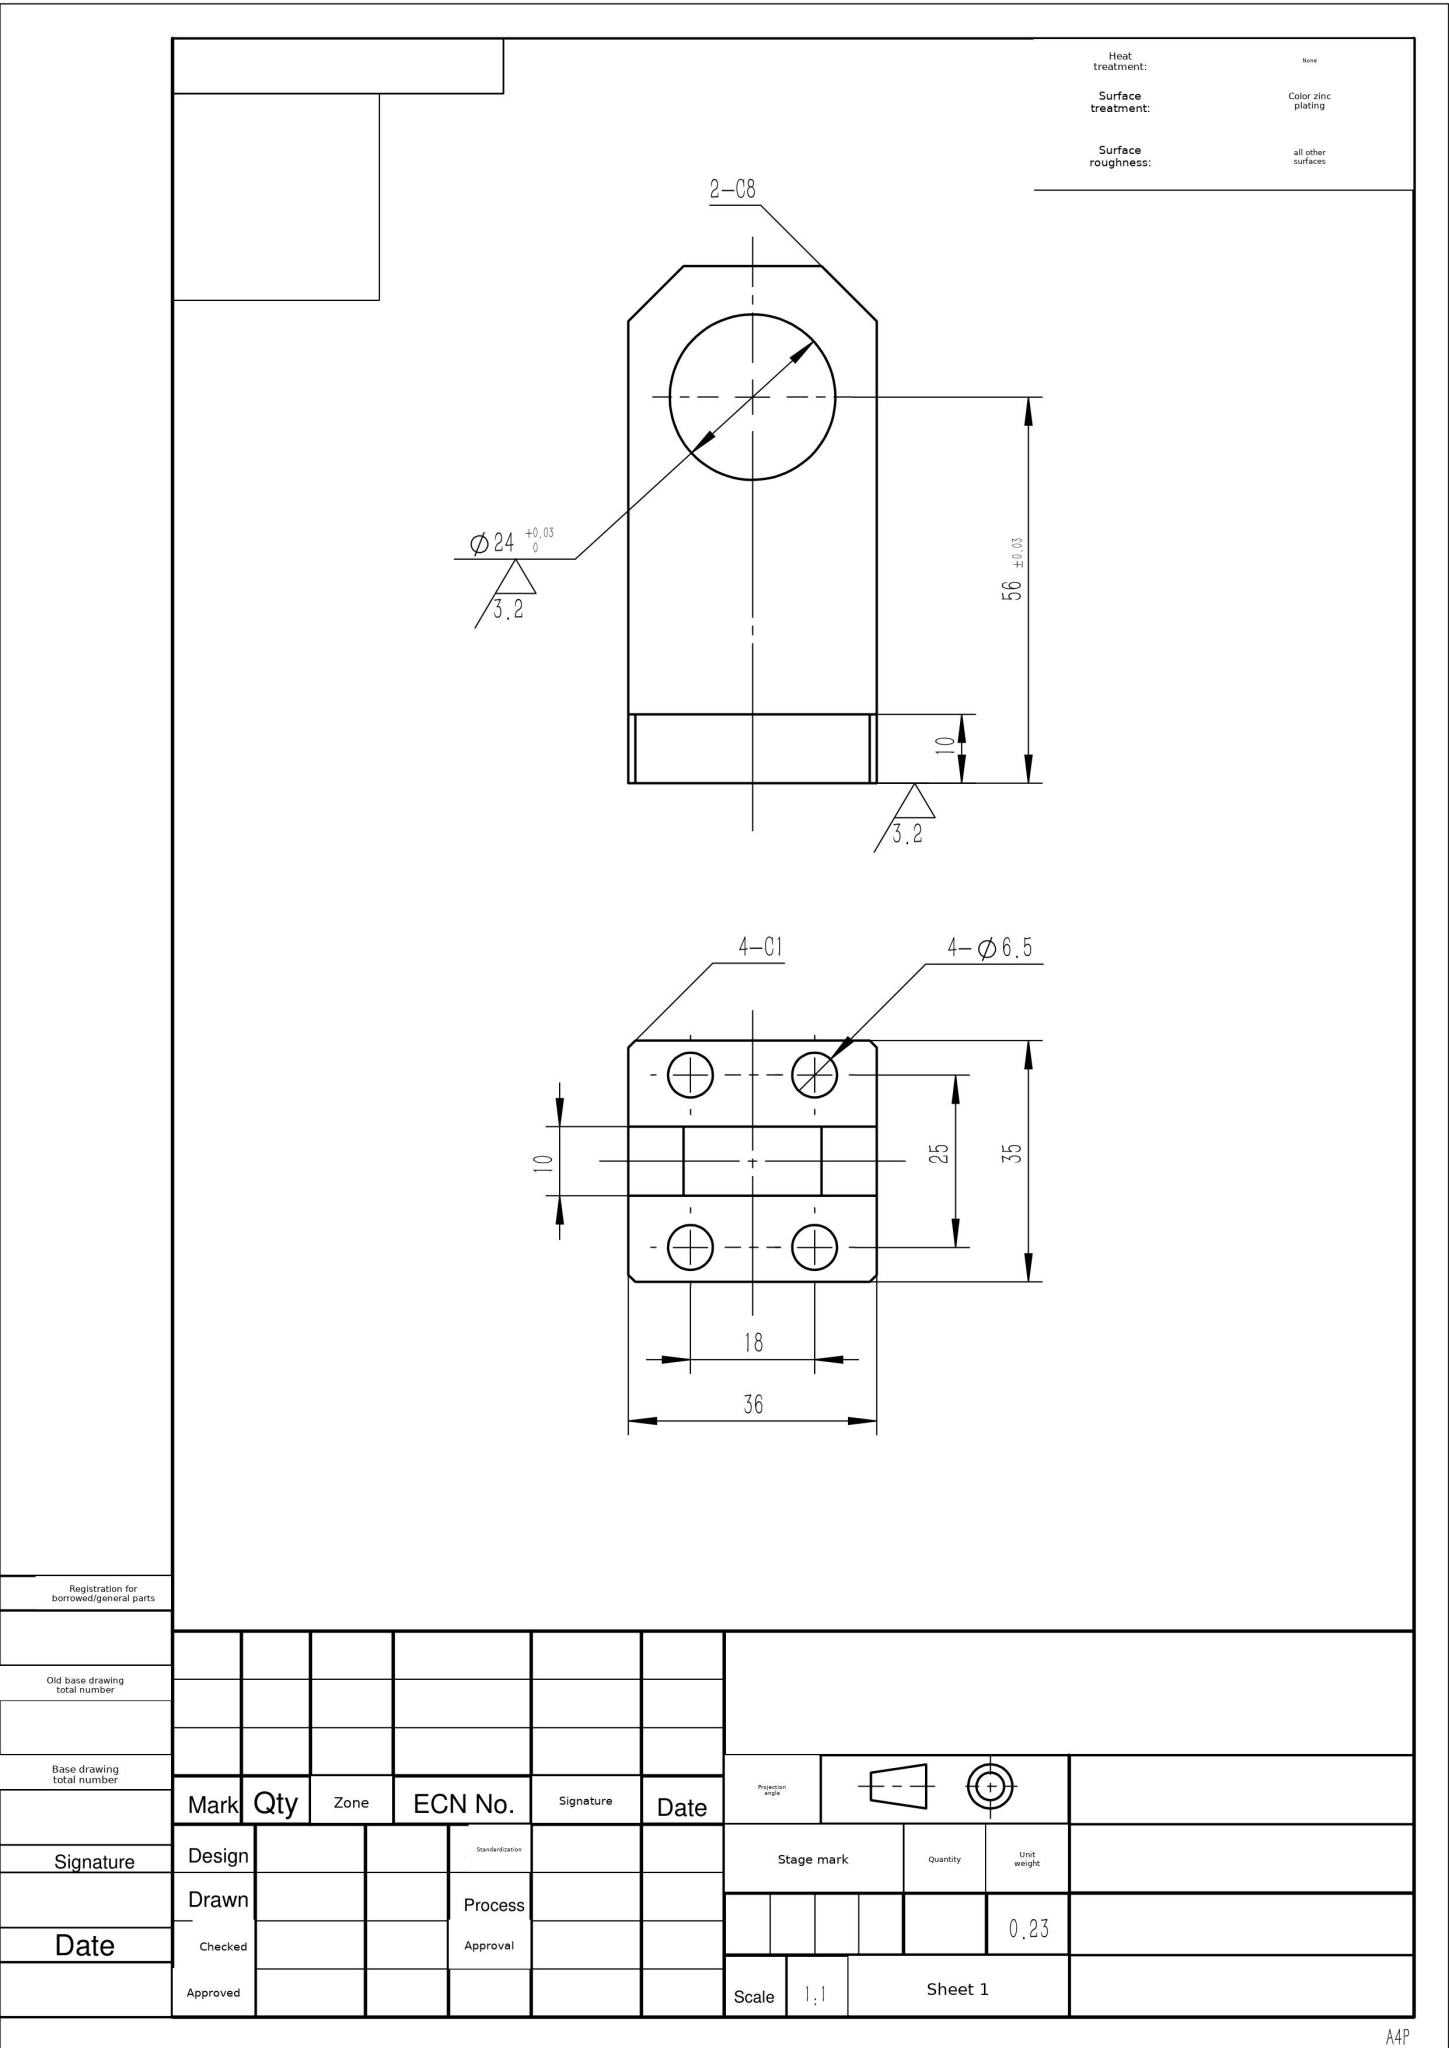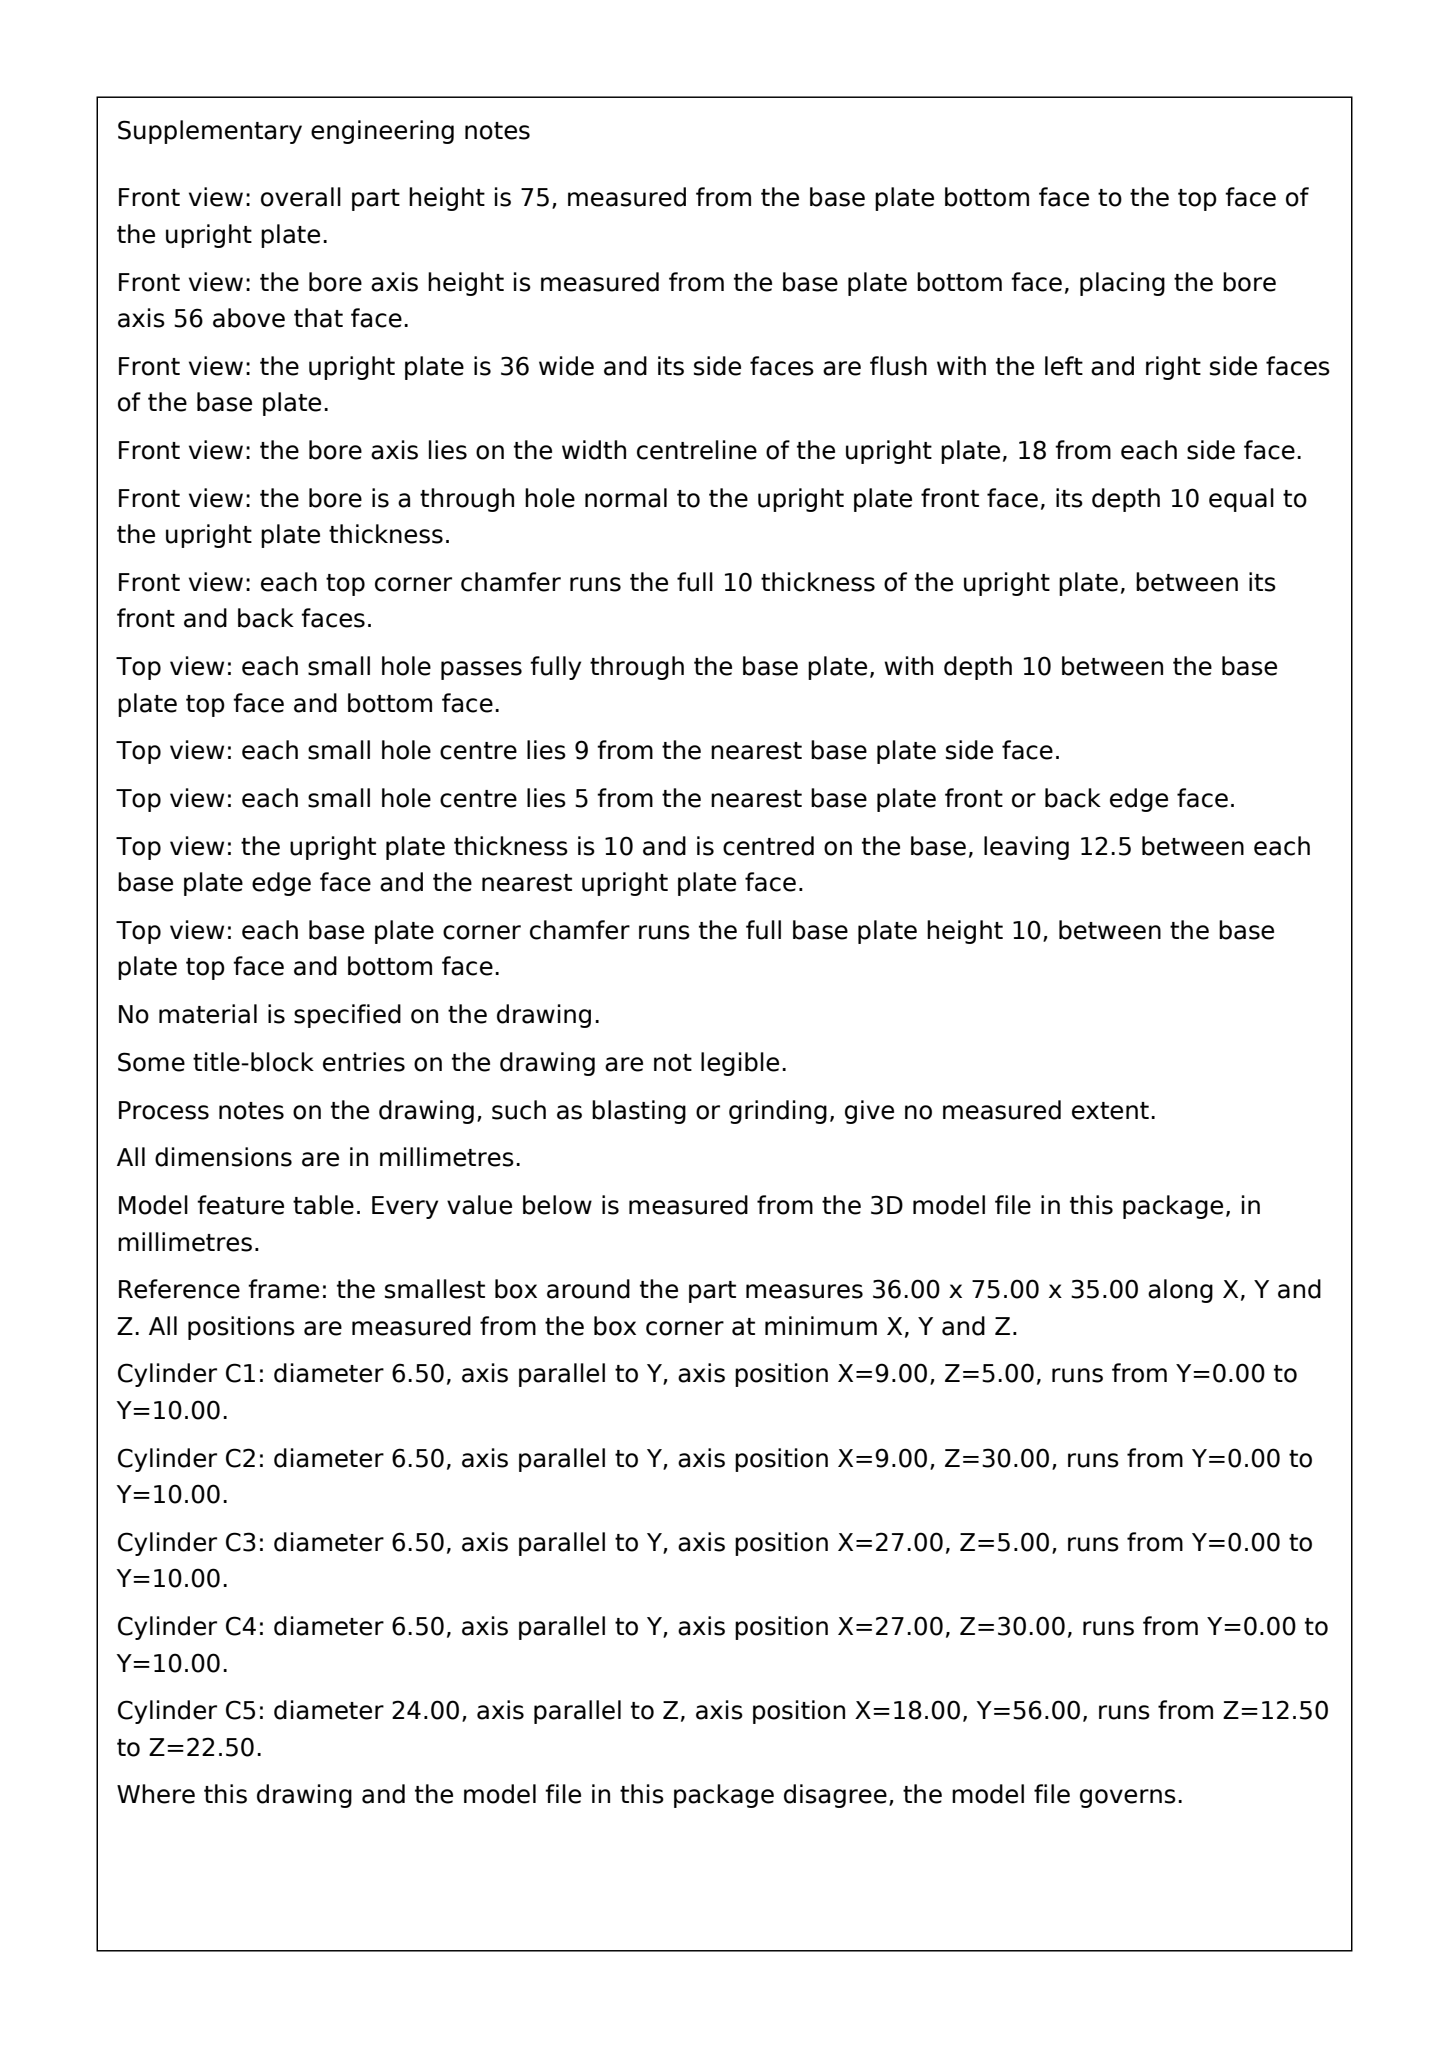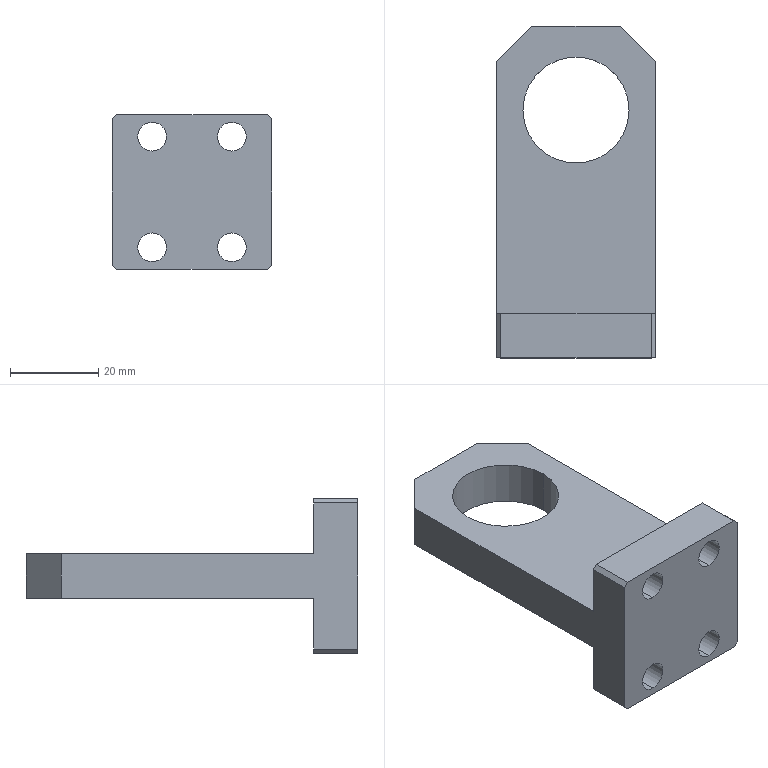Part | SolidWorks | mm | 1 solid | 26 faces | box 36 x 75 x 35 mm | volume 29489 mm3 | plane 16 | cylinder 10 | commonest cylinder face diameters 6.5 x8 24 x2
Drawing notes:
FRONT VIEW: OVERALL HT 75 FROM BOTTOM FACE TO TOP | from the solid: bbox_xyz Y=75; planes y=0 and y=75; hole axis at y=56
OVERALL HT 75 FROM BOTTOM FACE TO TOP OF Ø24 BOSS | from the solid: bbox_xyz y=75; base face y=0, top face plane y=75; Ø24 hole axis at y=56
build123d program:
from build123d import *

# Parameters (mm, degrees)
SKETCH1_W           = 36
SKETCH1_H           = 65
BOSS_EXTRUDE1_DEPTH = 5
SKETCH2_W           = 36
SKETCH2_H           = 35
BOSS_EXTRUDE2_DEPTH = 10
SKETCH3_R           = 12
CUT_EXTRUDE1_DEPTH  = 72.1
CHAMFER1_SIZE       = 8
SKETCH4_R           = 3.25
CUT_EXTRUDE2_DEPTH  = 70.68
CHAMFER2_SIZE       = 1


with BuildPart() as part:
    # Sketch1 → Boss-Extrude1 (new, symmetric)
    with BuildSketch(Plane.XY):
        with Locations((0, 32.5)):
            Rectangle(SKETCH1_W, SKETCH1_H)
    extrude(amount=BOSS_EXTRUDE1_DEPTH, both=True)

    # Sketch2 → Boss-Extrude2 (add)
    with BuildSketch(Plane.XZ):
        Rectangle(SKETCH2_W, SKETCH2_H)
    extrude(amount=BOSS_EXTRUDE2_DEPTH)

    # Sketch3 → Cut-Extrude1 (cut, through all)
    with BuildSketch(Plane(origin=(0, 0, -5), x_dir=(-1, 0, 0), z_dir=(0, 0, -1))):
        with Locations((0, 46)):
            Circle(SKETCH3_R)
    extrude(amount=-CUT_EXTRUDE1_DEPTH, mode=Mode.SUBTRACT)

    # Chamfer1
    chamfer1_edges = [part.edges().sort_by_distance(p)[0] for p in [
        (-18, 65, 0),
        (18, 65, 0),
    ]]
    chamfer(chamfer1_edges, length=CHAMFER1_SIZE)

    # Sketch4 → Cut-Extrude2 (cut, through all)
    with BuildSketch(Plane(origin=(0, 0, 0), x_dir=(1, 0, 0), z_dir=(0, 1, 0))):
        with Locations(Location((-9, -12.5, 0), (0, 0, 270))):
            Circle(SKETCH4_R)
        with Locations(Location((-9, 12.5, 0), (0, 0, 90))):
            Circle(SKETCH4_R)
        with Locations(Location((9, -12.5, 0), (0, 0, 270))):
            Circle(SKETCH4_R)
        with Locations(Location((9, 12.5, 0), (0, 0, 90))):
            Circle(SKETCH4_R)
    extrude(amount=-CUT_EXTRUDE2_DEPTH, mode=Mode.SUBTRACT)

    # Chamfer2
    chamfer2_edges = [part.edges().sort_by_distance(p)[0] for p in [
        (18, -5, -17.5),
        (18, -5, 17.5),
        (-18, -5, 17.5),
        (-18, -5, -17.5),
    ]]
    chamfer(chamfer2_edges, length=CHAMFER2_SIZE)


solid = part.part
STEP:
#1=CARTESIAN_POINT('',(9.,-10.,9.25));
#2=VERTEX_POINT('',#1);
#3=CARTESIAN_POINT('',(9.,-10.,15.75));
#4=VERTEX_POINT('',#3);
#5=CARTESIAN_POINT('',(9.,-10.,12.5));
#6=DIRECTION('',(0.,1.,0.));
#7=DIRECTION('',(0.,0.,1.));
#8=AXIS2_PLACEMENT_3D('',#5,#6,#7);
#9=CIRCLE('',#8,3.25);
#10=EDGE_CURVE('',#2,#4,#9,.T.);
#11=ORIENTED_EDGE('',*,*,#10,.F.);
#12=CARTESIAN_POINT('',(9.,0.,9.25));
#13=VERTEX_POINT('',#12);
#14=CARTESIAN_POINT('',(9.,-10.,9.25));
#15=DIRECTION('',(0.,1.,0.));
#16=VECTOR('',#15,1000.);
#17=LINE('',#14,#16);
#18=EDGE_CURVE('',#2,#13,#17,.T.);
#19=ORIENTED_EDGE('',*,*,#18,.T.);
#20=CARTESIAN_POINT('',(9.,0.,15.75));
#21=VERTEX_POINT('',#20);
#22=CARTESIAN_POINT('',(9.,0.,12.5));
#23=DIRECTION('',(0.,1.,0.));
#24=DIRECTION('',(0.,0.,1.));
#25=AXIS2_PLACEMENT_3D('',#22,#23,#24);
#26=CIRCLE('',#25,3.25);
#27=EDGE_CURVE('',#13,#21,#26,.T.);
#28=ORIENTED_EDGE('',*,*,#27,.T.);
#29=CARTESIAN_POINT('',(9.,-10.,15.75));
#30=DIRECTION('',(0.,1.,0.));
#31=VECTOR('',#30,1000.);
#32=LINE('',#29,#31);
#33=EDGE_CURVE('',#4,#21,#32,.T.);
#34=ORIENTED_EDGE('',*,*,#33,.F.);
#35=EDGE_LOOP('',(#11,#19,#28,#34));
#36=FACE_OUTER_BOUND('',#35,.T.);
#37=CARTESIAN_POINT('',(9.,-10.,12.5));
#38=DIRECTION('',(0.,1.,0.));
#39=DIRECTION('',(0.,0.,1.));
#40=AXIS2_PLACEMENT_3D('',#37,#38,#39);
#41=CYLINDRICAL_SURFACE('',#40,3.25);
#42=ADVANCED_FACE('',(#36),#41,.F.);
#43=CARTESIAN_POINT('',(-9.,-10.,-15.75));
#44=VERTEX_POINT('',#43);
#45=CARTESIAN_POINT('',(-9.,-10.,-9.25));
#46=VERTEX_POINT('',#45);
#47=CARTESIAN_POINT('',(-9.,-10.,-12.5));
#48=DIRECTION('',(0.,1.,0.));
#49=DIRECTION('',(0.,0.,-1.));
#50=AXIS2_PLACEMENT_3D('',#47,#48,#49);
#51=CIRCLE('',#50,3.25);
#52=EDGE_CURVE('',#44,#46,#51,.T.);
#53=ORIENTED_EDGE('',*,*,#52,.F.);
#54=CARTESIAN_POINT('',(-9.,0.,-15.75));
#55=VERTEX_POINT('',#54);
#56=CARTESIAN_POINT('',(-9.,-10.,-15.75));
#57=DIRECTION('',(0.,1.,0.));
#58=VECTOR('',#57,1000.);
#59=LINE('',#56,#58);
#60=EDGE_CURVE('',#44,#55,#59,.T.);
#61=ORIENTED_EDGE('',*,*,#60,.T.);
#62=CARTESIAN_POINT('',(-9.,0.,-9.25));
#63=VERTEX_POINT('',#62);
#64=CARTESIAN_POINT('',(-9.,0.,-12.5));
#65=DIRECTION('',(0.,1.,0.));
#66=DIRECTION('',(0.,0.,-1.));
#67=AXIS2_PLACEMENT_3D('',#64,#65,#66);
#68=CIRCLE('',#67,3.25);
#69=EDGE_CURVE('',#55,#63,#68,.T.);
#70=ORIENTED_EDGE('',*,*,#69,.T.);
#71=CARTESIAN_POINT('',(-9.,-10.,-9.25));
#72=DIRECTION('',(0.,1.,0.));
#73=VECTOR('',#72,1000.);
#74=LINE('',#71,#73);
#75=EDGE_CURVE('',#46,#63,#74,.T.);
#76=ORIENTED_EDGE('',*,*,#75,.F.);
#77=EDGE_LOOP('',(#53,#61,#70,#76));
#78=FACE_OUTER_BOUND('',#77,.T.);
#79=CARTESIAN_POINT('',(-9.,-10.,-12.5));
#80=DIRECTION('',(0.,1.,0.));
#81=DIRECTION('',(0.,0.,1.));
#82=AXIS2_PLACEMENT_3D('',#79,#80,#81);
#83=CYLINDRICAL_SURFACE('',#82,3.25);
#84=ADVANCED_FACE('',(#78),#83,.F.);
#85=CARTESIAN_POINT('',(9.,-10.,-15.75));
#86=VERTEX_POINT('',#85);
#87=CARTESIAN_POINT('',(9.,-10.,-9.25));
#88=VERTEX_POINT('',#87);
#89=CARTESIAN_POINT('',(9.,-10.,-12.5));
#90=DIRECTION('',(0.,1.,0.));
#91=DIRECTION('',(0.,0.,-1.));
#92=AXIS2_PLACEMENT_3D('',#89,#90,#91);
#93=CIRCLE('',#92,3.25);
#94=EDGE_CURVE('',#86,#88,#93,.T.);
#95=ORIENTED_EDGE('',*,*,#94,.F.);
#96=CARTESIAN_POINT('',(9.,0.,-15.75));
#97=VERTEX_POINT('',#96);
#98=CARTESIAN_POINT('',(9.,-10.,-15.75));
#99=DIRECTION('',(0.,1.,0.));
#100=VECTOR('',#99,1000.);
#101=LINE('',#98,#100);
#102=EDGE_CURVE('',#86,#97,#101,.T.);
#103=ORIENTED_EDGE('',*,*,#102,.T.);
#104=CARTESIAN_POINT('',(9.,0.,-9.25));
#105=VERTEX_POINT('',#104);
#106=CARTESIAN_POINT('',(9.,0.,-12.5));
#107=DIRECTION('',(0.,1.,0.));
#108=DIRECTION('',(0.,0.,-1.));
#109=AXIS2_PLACEMENT_3D('',#106,#107,#108);
#110=CIRCLE('',#109,3.25);
#111=EDGE_CURVE('',#97,#105,#110,.T.);
#112=ORIENTED_EDGE('',*,*,#111,.T.);
#113=CARTESIAN_POINT('',(9.,-10.,-9.25));
#114=DIRECTION('',(0.,1.,0.));
#115=VECTOR('',#114,1000.);
#116=LINE('',#113,#115);
#117=EDGE_CURVE('',#88,#105,#116,.T.);
#118=ORIENTED_EDGE('',*,*,#117,.F.);
#119=EDGE_LOOP('',(#95,#103,#112,#118));
#120=FACE_OUTER_BOUND('',#119,.T.);
#121=CARTESIAN_POINT('',(9.,-10.,-12.5));
#122=DIRECTION('',(0.,1.,0.));
#123=DIRECTION('',(0.,0.,1.));
#124=AXIS2_PLACEMENT_3D('',#121,#122,#123);
#125=CYLINDRICAL_SURFACE('',#124,3.25);
#126=ADVANCED_FACE('',(#120),#125,.F.);
#127=CARTESIAN_POINT('',(-9.,-10.,9.25));
#128=VERTEX_POINT('',#127);
#129=CARTESIAN_POINT('',(-9.,-10.,15.75));
#130=VERTEX_POINT('',#129);
#131=CARTESIAN_POINT('',(-9.,-10.,12.5));
#132=DIRECTION('',(0.,1.,0.));
#133=DIRECTION('',(0.,0.,1.));
#134=AXIS2_PLACEMENT_3D('',#131,#132,#133);
#135=CIRCLE('',#134,3.25);
#136=EDGE_CURVE('',#128,#130,#135,.T.);
#137=ORIENTED_EDGE('',*,*,#136,.F.);
#138=CARTESIAN_POINT('',(-9.,0.,9.25));
#139=VERTEX_POINT('',#138);
#140=CARTESIAN_POINT('',(-9.,-10.,9.25));
#141=DIRECTION('',(0.,1.,0.));
#142=VECTOR('',#141,1000.);
#143=LINE('',#140,#142);
#144=EDGE_CURVE('',#128,#139,#143,.T.);
#145=ORIENTED_EDGE('',*,*,#144,.T.);
#146=CARTESIAN_POINT('',(-9.,0.,15.75));
#147=VERTEX_POINT('',#146);
#148=CARTESIAN_POINT('',(-9.,0.,12.5));
#149=DIRECTION('',(0.,1.,0.));
#150=DIRECTION('',(0.,0.,1.));
#151=AXIS2_PLACEMENT_3D('',#148,#149,#150);
#152=CIRCLE('',#151,3.25);
#153=EDGE_CURVE('',#139,#147,#152,.T.);
#154=ORIENTED_EDGE('',*,*,#153,.T.);
#155=CARTESIAN_POINT('',(-9.,-10.,15.75));
#156=DIRECTION('',(0.,1.,0.));
#157=VECTOR('',#156,1000.);
#158=LINE('',#155,#157);
#159=EDGE_CURVE('',#130,#147,#158,.T.);
#160=ORIENTED_EDGE('',*,*,#159,.F.);
#161=EDGE_LOOP('',(#137,#145,#154,#160));
#162=FACE_OUTER_BOUND('',#161,.T.);
#163=CARTESIAN_POINT('',(-9.,-10.,12.5));
#164=DIRECTION('',(0.,1.,0.));
#165=DIRECTION('',(0.,0.,1.));
#166=AXIS2_PLACEMENT_3D('',#163,#164,#165);
#167=CYLINDRICAL_SURFACE('',#166,3.25);
#168=ADVANCED_FACE('',(#162),#167,.F.);
#169=CARTESIAN_POINT('',(-12.,46.,5.));
#170=VERTEX_POINT('',#169);
#171=CARTESIAN_POINT('',(12.,46.,5.));
#172=VERTEX_POINT('',#171);
#173=CARTESIAN_POINT('',(0.,46.,5.));
#174=DIRECTION('',(0.,0.,1.));
#175=DIRECTION('',(1.,0.,0.));
#176=AXIS2_PLACEMENT_3D('',#173,#174,#175);
#177=CIRCLE('',#176,12.);
#178=EDGE_CURVE('',#170,#172,#177,.T.);
#179=ORIENTED_EDGE('',*,*,#178,.T.);
#180=CARTESIAN_POINT('',(12.,46.,-5.));
#181=VERTEX_POINT('',#180);
#182=CARTESIAN_POINT('',(12.,46.,17.5));
#183=DIRECTION('',(0.,0.,-1.));
#184=VECTOR('',#183,1000.);
#185=LINE('',#182,#184);
#186=EDGE_CURVE('',#172,#181,#185,.T.);
#187=ORIENTED_EDGE('',*,*,#186,.T.);
#188=CARTESIAN_POINT('',(-12.,46.,-5.));
#189=VERTEX_POINT('',#188);
#190=CARTESIAN_POINT('',(0.,46.,-5.));
#191=DIRECTION('',(0.,0.,-1.));
#192=DIRECTION('',(-1.,0.,0.));
#193=AXIS2_PLACEMENT_3D('',#190,#191,#192);
#194=CIRCLE('',#193,12.);
#195=EDGE_CURVE('',#181,#189,#194,.T.);
#196=ORIENTED_EDGE('',*,*,#195,.T.);
#197=CARTESIAN_POINT('',(-12.,46.,17.5));
#198=DIRECTION('',(0.,0.,-1.));
#199=VECTOR('',#198,1000.);
#200=LINE('',#197,#199);
#201=EDGE_CURVE('',#170,#189,#200,.T.);
#202=ORIENTED_EDGE('',*,*,#201,.F.);
#203=EDGE_LOOP('',(#179,#187,#196,#202));
#204=FACE_OUTER_BOUND('',#203,.T.);
#205=CARTESIAN_POINT('',(0.,46.,17.5));
#206=DIRECTION('',(0.,0.,-1.));
#207=DIRECTION('',(-1.,0.,0.));
#208=AXIS2_PLACEMENT_3D('',#205,#206,#207);
#209=CYLINDRICAL_SURFACE('',#208,12.);
#210=ADVANCED_FACE('',(#204),#209,.F.);
#211=CARTESIAN_POINT('',(-18.,0.,-5.));
#212=VERTEX_POINT('',#211);
#213=CARTESIAN_POINT('',(-18.,0.,-16.5));
#214=VERTEX_POINT('',#213);
#215=CARTESIAN_POINT('',(-18.,0.,-17.5));
#216=DIRECTION('',(0.,0.,-1.));
#217=VECTOR('',#216,1000.);
#218=LINE('',#215,#217);
#219=EDGE_CURVE('',#212,#214,#218,.T.);
#220=ORIENTED_EDGE('',*,*,#219,.T.);
#221=CARTESIAN_POINT('',(-18.,-10.,-16.5));
#222=VERTEX_POINT('',#221);
#223=CARTESIAN_POINT('',(-18.,65.,-16.5));
#224=DIRECTION('',(0.,-1.,0.));
#225=VECTOR('',#224,1000.);
#226=LINE('',#223,#225);
#227=EDGE_CURVE('',#214,#222,#226,.T.);
#228=ORIENTED_EDGE('',*,*,#227,.T.);
#229=CARTESIAN_POINT('',(-18.,-10.,16.5));
#230=VERTEX_POINT('',#229);
#231=CARTESIAN_POINT('',(-18.,-10.,-17.5));
#232=DIRECTION('',(0.,0.,-1.));
#233=VECTOR('',#232,1000.);
#234=LINE('',#231,#233);
#235=EDGE_CURVE('',#230,#222,#234,.T.);
#236=ORIENTED_EDGE('',*,*,#235,.F.);
#237=CARTESIAN_POINT('',(-18.,0.,16.5));
#238=VERTEX_POINT('',#237);
#239=CARTESIAN_POINT('',(-18.,65.,16.5));
#240=DIRECTION('',(-0.,1.,0.));
#241=VECTOR('',#240,1000.);
#242=LINE('',#239,#241);
#243=EDGE_CURVE('',#230,#238,#242,.T.);
#244=ORIENTED_EDGE('',*,*,#243,.T.);
#245=CARTESIAN_POINT('',(-18.,0.,5.));
#246=VERTEX_POINT('',#245);
#247=CARTESIAN_POINT('',(-18.,0.,-17.5));
#248=DIRECTION('',(0.,0.,-1.));
#249=VECTOR('',#248,1000.);
#250=LINE('',#247,#249);
#251=EDGE_CURVE('',#238,#246,#250,.T.);
#252=ORIENTED_EDGE('',*,*,#251,.T.);
#253=CARTESIAN_POINT('',(-18.,57.,5.));
#254=VERTEX_POINT('',#253);
#255=CARTESIAN_POINT('',(-18.,65.,5.));
#256=DIRECTION('',(0.,-1.,0.));
#257=VECTOR('',#256,1000.);
#258=LINE('',#255,#257);
#259=EDGE_CURVE('',#254,#246,#258,.T.);
#260=ORIENTED_EDGE('',*,*,#259,.F.);
#261=CARTESIAN_POINT('',(-18.,57.,-5.));
#262=VERTEX_POINT('',#261);
#263=CARTESIAN_POINT('',(-18.,57.,5.));
#264=DIRECTION('',(0.,0.,-1.));
#265=VECTOR('',#264,1000.);
#266=LINE('',#263,#265);
#267=EDGE_CURVE('',#254,#262,#266,.T.);
#268=ORIENTED_EDGE('',*,*,#267,.T.);
#269=CARTESIAN_POINT('',(-18.,65.,-5.));
#270=DIRECTION('',(0.,-1.,0.));
#271=VECTOR('',#270,1000.);
#272=LINE('',#269,#271);
#273=EDGE_CURVE('',#262,#212,#272,.T.);
#274=ORIENTED_EDGE('',*,*,#273,.T.);
#275=EDGE_LOOP('',(#220,#228,#236,#244,#252,#260,#268,#274));
#276=FACE_OUTER_BOUND('',#275,.T.);
#277=CARTESIAN_POINT('',(-18.,65.,5.));
#278=DIRECTION('',(1.,0.,0.));
#279=DIRECTION('',(-0.,1.,0.));
#280=AXIS2_PLACEMENT_3D('',#277,#278,#279);
#281=PLANE('',#280);
#282=ADVANCED_FACE('',(#276),#281,.F.);
#283=CARTESIAN_POINT('',(18.,-10.,-16.5));
#284=VERTEX_POINT('',#283);
#285=CARTESIAN_POINT('',(18.,-10.,16.5));
#286=VERTEX_POINT('',#285);
#287=CARTESIAN_POINT('',(18.,-10.,-17.5));
#288=DIRECTION('',(0.,0.,1.));
#289=VECTOR('',#288,1000.);
#290=LINE('',#287,#289);
#291=EDGE_CURVE('',#284,#286,#290,.T.);
#292=ORIENTED_EDGE('',*,*,#291,.F.);
#293=CARTESIAN_POINT('',(18.,0.,-16.5));
#294=VERTEX_POINT('',#293);
#295=CARTESIAN_POINT('',(18.,65.,-16.5));
#296=DIRECTION('',(0.,1.,0.));
#297=VECTOR('',#296,1000.);
#298=LINE('',#295,#297);
#299=EDGE_CURVE('',#284,#294,#298,.T.);
#300=ORIENTED_EDGE('',*,*,#299,.T.);
#301=CARTESIAN_POINT('',(18.,0.,-5.));
#302=VERTEX_POINT('',#301);
#303=CARTESIAN_POINT('',(18.,0.,-17.5));
#304=DIRECTION('',(0.,0.,1.));
#305=VECTOR('',#304,1000.);
#306=LINE('',#303,#305);
#307=EDGE_CURVE('',#294,#302,#306,.T.);
#308=ORIENTED_EDGE('',*,*,#307,.T.);
#309=CARTESIAN_POINT('',(18.,57.,-5.));
#310=VERTEX_POINT('',#309);
#311=CARTESIAN_POINT('',(18.,65.,-5.));
#312=DIRECTION('',(0.,1.,0.));
#313=VECTOR('',#312,1000.);
#314=LINE('',#311,#313);
#315=EDGE_CURVE('',#302,#310,#314,.T.);
#316=ORIENTED_EDGE('',*,*,#315,.T.);
#317=CARTESIAN_POINT('',(18.,57.,5.));
#318=VERTEX_POINT('',#317);
#319=CARTESIAN_POINT('',(18.,57.,5.));
#320=DIRECTION('',(0.,0.,1.));
#321=VECTOR('',#320,1000.);
#322=LINE('',#319,#321);
#323=EDGE_CURVE('',#310,#318,#322,.T.);
#324=ORIENTED_EDGE('',*,*,#323,.T.);
#325=CARTESIAN_POINT('',(18.,0.,5.));
#326=VERTEX_POINT('',#325);
#327=CARTESIAN_POINT('',(18.,65.,5.));
#328=DIRECTION('',(0.,1.,0.));
#329=VECTOR('',#328,1000.);
#330=LINE('',#327,#329);
#331=EDGE_CURVE('',#326,#318,#330,.T.);
#332=ORIENTED_EDGE('',*,*,#331,.F.);
#333=CARTESIAN_POINT('',(18.,0.,16.5));
#334=VERTEX_POINT('',#333);
#335=CARTESIAN_POINT('',(18.,0.,-17.5));
#336=DIRECTION('',(0.,0.,1.));
#337=VECTOR('',#336,1000.);
#338=LINE('',#335,#337);
#339=EDGE_CURVE('',#326,#334,#338,.T.);
#340=ORIENTED_EDGE('',*,*,#339,.T.);
#341=CARTESIAN_POINT('',(18.,65.,16.5));
#342=DIRECTION('',(-0.,-1.,0.));
#343=VECTOR('',#342,1000.);
#344=LINE('',#341,#343);
#345=EDGE_CURVE('',#334,#286,#344,.T.);
#346=ORIENTED_EDGE('',*,*,#345,.T.);
#347=EDGE_LOOP('',(#292,#300,#308,#316,#324,#332,#340,#346));
#348=FACE_OUTER_BOUND('',#347,.T.);
#349=CARTESIAN_POINT('',(18.,65.,5.));
#350=DIRECTION('',(-1.,0.,0.));
#351=DIRECTION('',(-0.,-1.,0.));
#352=AXIS2_PLACEMENT_3D('',#349,#350,#351);
#353=PLANE('',#352);
#354=ADVANCED_FACE('',(#348),#353,.F.);
#355=CARTESIAN_POINT('',(10.,65.,-5.));
#356=VERTEX_POINT('',#355);
#357=CARTESIAN_POINT('',(-10.,65.,-5.));
#358=VERTEX_POINT('',#357);
#359=CARTESIAN_POINT('',(18.,65.,-5.));
#360=DIRECTION('',(-1.,0.,0.));
#361=VECTOR('',#360,1000.);
#362=LINE('',#359,#361);
#363=EDGE_CURVE('',#356,#358,#362,.T.);
#364=ORIENTED_EDGE('',*,*,#363,.T.);
#365=CARTESIAN_POINT('',(-10.,65.,5.));
#366=VERTEX_POINT('',#365);
#367=CARTESIAN_POINT('',(-10.,65.,5.));
#368=DIRECTION('',(0.,0.,1.));
#369=VECTOR('',#368,1000.);
#370=LINE('',#367,#369);
#371=EDGE_CURVE('',#358,#366,#370,.T.);
#372=ORIENTED_EDGE('',*,*,#371,.T.);
#373=CARTESIAN_POINT('',(10.,65.,5.));
#374=VERTEX_POINT('',#373);
#375=CARTESIAN_POINT('',(18.,65.,5.));
#376=DIRECTION('',(-1.,0.,0.));
#377=VECTOR('',#376,1000.);
#378=LINE('',#375,#377);
#379=EDGE_CURVE('',#374,#366,#378,.T.);
#380=ORIENTED_EDGE('',*,*,#379,.F.);
#381=CARTESIAN_POINT('',(10.,65.,5.));
#382=DIRECTION('',(0.,0.,-1.));
#383=VECTOR('',#382,1000.);
#384=LINE('',#381,#383);
#385=EDGE_CURVE('',#374,#356,#384,.T.);
#386=ORIENTED_EDGE('',*,*,#385,.T.);
#387=EDGE_LOOP('',(#364,#372,#380,#386));
#388=FACE_OUTER_BOUND('',#387,.T.);
#389=CARTESIAN_POINT('',(18.,65.,5.));
#390=DIRECTION('',(0.,-1.,0.));
#391=DIRECTION('',(0.,0.,-1.));
#392=AXIS2_PLACEMENT_3D('',#389,#390,#391);
#393=PLANE('',#392);
#394=ADVANCED_FACE('',(#388),#393,.F.);
#395=ORIENTED_EDGE('',*,*,#178,.F.);
#396=CARTESIAN_POINT('',(0.,46.,5.));
#397=DIRECTION('',(0.,0.,1.));
#398=DIRECTION('',(1.,0.,0.));
#399=AXIS2_PLACEMENT_3D('',#396,#397,#398);
#400=CIRCLE('',#399,12.);
#401=EDGE_CURVE('',#172,#170,#400,.T.);
#402=ORIENTED_EDGE('',*,*,#401,.F.);
#403=EDGE_LOOP('',(#395,#402));
#404=FACE_BOUND('',#403,.T.);
#405=ORIENTED_EDGE('',*,*,#379,.T.);
#406=CARTESIAN_POINT('',(-37.5,37.5,5.));
#407=DIRECTION('',(-0.7071,-0.7071,0.));
#408=VECTOR('',#407,1000.);
#409=LINE('',#406,#408);
#410=EDGE_CURVE('',#366,#254,#409,.T.);
#411=ORIENTED_EDGE('',*,*,#410,.T.);
#412=ORIENTED_EDGE('',*,*,#259,.T.);
#413=CARTESIAN_POINT('',(-18.,0.,5.));
#414=DIRECTION('',(1.,0.,0.));
#415=VECTOR('',#414,1000.);
#416=LINE('',#413,#415);
#417=EDGE_CURVE('',#246,#326,#416,.T.);
#418=ORIENTED_EDGE('',*,*,#417,.T.);
#419=ORIENTED_EDGE('',*,*,#331,.T.);
#420=CARTESIAN_POINT('',(37.5,37.5,5.));
#421=DIRECTION('',(-0.7071,0.7071,0.));
#422=VECTOR('',#421,1000.);
#423=LINE('',#420,#422);
#424=EDGE_CURVE('',#318,#374,#423,.T.);
#425=ORIENTED_EDGE('',*,*,#424,.T.);
#426=EDGE_LOOP('',(#405,#411,#412,#418,#419,#425));
#427=FACE_OUTER_BOUND('',#426,.T.);
#428=CARTESIAN_POINT('',(0.,0.,5.));
#429=DIRECTION('',(0.,0.,1.));
#430=DIRECTION('',(1.,0.,0.));
#431=AXIS2_PLACEMENT_3D('',#428,#429,#430);
#432=PLANE('',#431);
#433=ADVANCED_FACE('',(#404,#427),#432,.T.);
#434=CARTESIAN_POINT('',(0.,46.,-5.));
#435=DIRECTION('',(0.,0.,-1.));
#436=DIRECTION('',(-1.,0.,0.));
#437=AXIS2_PLACEMENT_3D('',#434,#435,#436);
#438=CIRCLE('',#437,12.);
#439=EDGE_CURVE('',#189,#181,#438,.T.);
#440=ORIENTED_EDGE('',*,*,#439,.F.);
#441=ORIENTED_EDGE('',*,*,#195,.F.);
#442=EDGE_LOOP('',(#440,#441));
#443=FACE_BOUND('',#442,.T.);
#444=ORIENTED_EDGE('',*,*,#273,.F.);
#445=CARTESIAN_POINT('',(-18.,57.,-5.));
#446=DIRECTION('',(0.7071,0.7071,0.));
#447=VECTOR('',#446,1000.);
#448=LINE('',#445,#447);
#449=EDGE_CURVE('',#262,#358,#448,.T.);
#450=ORIENTED_EDGE('',*,*,#449,.T.);
#451=ORIENTED_EDGE('',*,*,#363,.F.);
#452=CARTESIAN_POINT('',(10.,65.,-5.));
#453=DIRECTION('',(0.7071,-0.7071,0.));
#454=VECTOR('',#453,1000.);
#455=LINE('',#452,#454);
#456=EDGE_CURVE('',#356,#310,#455,.T.);
#457=ORIENTED_EDGE('',*,*,#456,.T.);
#458=ORIENTED_EDGE('',*,*,#315,.F.);
#459=CARTESIAN_POINT('',(-18.,0.,-5.));
#460=DIRECTION('',(1.,0.,0.));
#461=VECTOR('',#460,1000.);
#462=LINE('',#459,#461);
#463=EDGE_CURVE('',#212,#302,#462,.T.);
#464=ORIENTED_EDGE('',*,*,#463,.F.);
#465=EDGE_LOOP('',(#444,#450,#451,#457,#458,#464));
#466=FACE_OUTER_BOUND('',#465,.T.);
#467=CARTESIAN_POINT('',(0.,0.,-5.));
#468=DIRECTION('',(0.,0.,1.));
#469=DIRECTION('',(1.,0.,0.));
#470=AXIS2_PLACEMENT_3D('',#467,#468,#469);
#471=PLANE('',#470);
#472=ADVANCED_FACE('',(#443,#466),#471,.F.);
#473=CARTESIAN_POINT('',(9.,0.,12.5));
#474=DIRECTION('',(0.,1.,0.));
#475=DIRECTION('',(0.,0.,1.));
#476=AXIS2_PLACEMENT_3D('',#473,#474,#475);
#477=CIRCLE('',#476,3.25);
#478=EDGE_CURVE('',#21,#13,#477,.T.);
#479=ORIENTED_EDGE('',*,*,#478,.F.);
#480=ORIENTED_EDGE('',*,*,#27,.F.);
#481=EDGE_LOOP('',(#479,#480));
#482=FACE_BOUND('',#481,.T.);
#483=CARTESIAN_POINT('',(-9.,0.,12.5));
#484=DIRECTION('',(0.,1.,0.));
#485=DIRECTION('',(0.,0.,1.));
#486=AXIS2_PLACEMENT_3D('',#483,#484,#485);
#487=CIRCLE('',#486,3.25);
#488=EDGE_CURVE('',#147,#139,#487,.T.);
#489=ORIENTED_EDGE('',*,*,#488,.F.);
#490=ORIENTED_EDGE('',*,*,#153,.F.);
#491=EDGE_LOOP('',(#489,#490));
#492=FACE_BOUND('',#491,.T.);
#493=ORIENTED_EDGE('',*,*,#251,.F.);
#494=CARTESIAN_POINT('',(-17.,0.,17.5));
#495=VERTEX_POINT('',#494);
#496=CARTESIAN_POINT('',(-17.25,0.,17.25));
#497=DIRECTION('',(0.7071,0.,0.7071));
#498=VECTOR('',#497,1000.);
#499=LINE('',#496,#498);
#500=EDGE_CURVE('',#238,#495,#499,.T.);
#501=ORIENTED_EDGE('',*,*,#500,.T.);
#502=CARTESIAN_POINT('',(17.,0.,17.5));
#503=VERTEX_POINT('',#502);
#504=CARTESIAN_POINT('',(-18.,0.,17.5));
#505=DIRECTION('',(-1.,0.,0.));
#506=VECTOR('',#505,1000.);
#507=LINE('',#504,#506);
#508=EDGE_CURVE('',#503,#495,#507,.T.);
#509=ORIENTED_EDGE('',*,*,#508,.F.);
#510=CARTESIAN_POINT('',(17.25,0.,17.25));
#511=DIRECTION('',(0.7071,0.,-0.7071));
#512=VECTOR('',#511,1000.);
#513=LINE('',#510,#512);
#514=EDGE_CURVE('',#503,#334,#513,.T.);
#515=ORIENTED_EDGE('',*,*,#514,.T.);
#516=ORIENTED_EDGE('',*,*,#339,.F.);
#517=ORIENTED_EDGE('',*,*,#417,.F.);
#518=EDGE_LOOP('',(#493,#501,#509,#515,#516,#517));
#519=FACE_OUTER_BOUND('',#518,.T.);
#520=CARTESIAN_POINT('',(0.,0.,0.));
#521=DIRECTION('',(0.,1.,0.));
#522=DIRECTION('',(0.,0.,1.));
#523=AXIS2_PLACEMENT_3D('',#520,#521,#522);
#524=PLANE('',#523);
#525=ADVANCED_FACE('',(#482,#492,#519),#524,.T.);
#526=ORIENTED_EDGE('',*,*,#508,.T.);
#527=CARTESIAN_POINT('',(-17.,-10.,17.5));
#528=VERTEX_POINT('',#527);
#529=CARTESIAN_POINT('',(-17.,-10.,17.5));
#530=DIRECTION('',(0.,-1.,0.));
#531=VECTOR('',#530,1000.);
#532=LINE('',#529,#531);
#533=EDGE_CURVE('',#495,#528,#532,.T.);
#534=ORIENTED_EDGE('',*,*,#533,.T.);
#535=CARTESIAN_POINT('',(17.,-10.,17.5));
#536=VERTEX_POINT('',#535);
#537=CARTESIAN_POINT('',(-18.,-10.,17.5));
#538=DIRECTION('',(-1.,0.,0.));
#539=VECTOR('',#538,1000.);
#540=LINE('',#537,#539);
#541=EDGE_CURVE('',#536,#528,#540,.T.);
#542=ORIENTED_EDGE('',*,*,#541,.F.);
#543=CARTESIAN_POINT('',(17.,-10.,17.5));
#544=DIRECTION('',(0.,1.,0.));
#545=VECTOR('',#544,1000.);
#546=LINE('',#543,#545);
#547=EDGE_CURVE('',#536,#503,#546,.T.);
#548=ORIENTED_EDGE('',*,*,#547,.T.);
#549=EDGE_LOOP('',(#526,#534,#542,#548));
#550=FACE_OUTER_BOUND('',#549,.T.);
#551=CARTESIAN_POINT('',(-18.,-10.,17.5));
#552=DIRECTION('',(0.,0.,-1.));
#553=DIRECTION('',(-1.,0.,0.));
#554=AXIS2_PLACEMENT_3D('',#551,#552,#553);
#555=PLANE('',#554);
#556=ADVANCED_FACE('',(#550),#555,.F.);
#557=CARTESIAN_POINT('',(-17.,0.,-17.5));
#558=VERTEX_POINT('',#557);
#559=CARTESIAN_POINT('',(17.,0.,-17.5));
#560=VERTEX_POINT('',#559);
#561=CARTESIAN_POINT('',(-18.,0.,-17.5));
#562=DIRECTION('',(1.,0.,0.));
#563=VECTOR('',#562,1000.);
#564=LINE('',#561,#563);
#565=EDGE_CURVE('',#558,#560,#564,.T.);
#566=ORIENTED_EDGE('',*,*,#565,.T.);
#567=CARTESIAN_POINT('',(17.,-10.,-17.5));
#568=VERTEX_POINT('',#567);
#569=CARTESIAN_POINT('',(17.,-10.,-17.5));
#570=DIRECTION('',(-0.,-1.,0.));
#571=VECTOR('',#570,1000.);
#572=LINE('',#569,#571);
#573=EDGE_CURVE('',#560,#568,#572,.T.);
#574=ORIENTED_EDGE('',*,*,#573,.T.);
#575=CARTESIAN_POINT('',(-17.,-10.,-17.5));
#576=VERTEX_POINT('',#575);
#577=CARTESIAN_POINT('',(-18.,-10.,-17.5));
#578=DIRECTION('',(1.,0.,0.));
#579=VECTOR('',#578,1000.);
#580=LINE('',#577,#579);
#581=EDGE_CURVE('',#576,#568,#580,.T.);
#582=ORIENTED_EDGE('',*,*,#581,.F.);
#583=CARTESIAN_POINT('',(-17.,-10.,-17.5));
#584=DIRECTION('',(-0.,1.,0.));
#585=VECTOR('',#584,1000.);
#586=LINE('',#583,#585);
#587=EDGE_CURVE('',#576,#558,#586,.T.);
#588=ORIENTED_EDGE('',*,*,#587,.T.);
#589=EDGE_LOOP('',(#566,#574,#582,#588));
#590=FACE_OUTER_BOUND('',#589,.T.);
#591=CARTESIAN_POINT('',(-18.,-10.,-17.5));
#592=DIRECTION('',(0.,0.,1.));
#593=DIRECTION('',(1.,0.,0.));
#594=AXIS2_PLACEMENT_3D('',#591,#592,#593);
#595=PLANE('',#594);
#596=ADVANCED_FACE('',(#590),#595,.F.);
#597=CARTESIAN_POINT('',(-9.,-10.,-12.5));
#598=DIRECTION('',(0.,1.,0.));
#599=DIRECTION('',(0.,0.,-1.));
#600=AXIS2_PLACEMENT_3D('',#597,#598,#599);
#601=CIRCLE('',#600,3.25);
#602=EDGE_CURVE('',#46,#44,#601,.T.);
#603=ORIENTED_EDGE('',*,*,#602,.T.);
#604=ORIENTED_EDGE('',*,*,#52,.T.);
#605=EDGE_LOOP('',(#603,#604));
#606=FACE_BOUND('',#605,.T.);
#607=CARTESIAN_POINT('',(9.,-10.,12.5));
#608=DIRECTION('',(0.,1.,0.));
#609=DIRECTION('',(0.,0.,1.));
#610=AXIS2_PLACEMENT_3D('',#607,#608,#609);
#611=CIRCLE('',#610,3.25);
#612=EDGE_CURVE('',#4,#2,#611,.T.);
#613=ORIENTED_EDGE('',*,*,#612,.T.);
#614=ORIENTED_EDGE('',*,*,#10,.T.);
#615=EDGE_LOOP('',(#613,#614));
#616=FACE_BOUND('',#615,.T.);
#617=CARTESIAN_POINT('',(9.,-10.,-12.5));
#618=DIRECTION('',(0.,1.,0.));
#619=DIRECTION('',(0.,0.,-1.));
#620=AXIS2_PLACEMENT_3D('',#617,#618,#619);
#621=CIRCLE('',#620,3.25);
#622=EDGE_CURVE('',#88,#86,#621,.T.);
#623=ORIENTED_EDGE('',*,*,#622,.T.);
#624=ORIENTED_EDGE('',*,*,#94,.T.);
#625=EDGE_LOOP('',(#623,#624));
#626=FACE_BOUND('',#625,.T.);
#627=CARTESIAN_POINT('',(-9.,-10.,12.5));
#628=DIRECTION('',(0.,1.,0.));
#629=DIRECTION('',(0.,0.,1.));
#630=AXIS2_PLACEMENT_3D('',#627,#628,#629);
#631=CIRCLE('',#630,3.25);
#632=EDGE_CURVE('',#130,#128,#631,.T.);
#633=ORIENTED_EDGE('',*,*,#632,.T.);
#634=ORIENTED_EDGE('',*,*,#136,.T.);
#635=EDGE_LOOP('',(#633,#634));
#636=FACE_BOUND('',#635,.T.);
#637=ORIENTED_EDGE('',*,*,#581,.T.);
#638=CARTESIAN_POINT('',(18.,-10.,-16.5));
#639=DIRECTION('',(0.7071,0.,0.7071));
#640=VECTOR('',#639,1000.);
#641=LINE('',#638,#640);
#642=EDGE_CURVE('',#568,#284,#641,.T.);
#643=ORIENTED_EDGE('',*,*,#642,.T.);
#644=ORIENTED_EDGE('',*,*,#291,.T.);
#645=CARTESIAN_POINT('',(17.,-10.,17.5));
#646=DIRECTION('',(-0.7071,0.,0.7071));
#647=VECTOR('',#646,1000.);
#648=LINE('',#645,#647);
#649=EDGE_CURVE('',#286,#536,#648,.T.);
#650=ORIENTED_EDGE('',*,*,#649,.T.);
#651=ORIENTED_EDGE('',*,*,#541,.T.);
#652=CARTESIAN_POINT('',(-18.,-10.,16.5));
#653=DIRECTION('',(-0.7071,0.,-0.7071));
#654=VECTOR('',#653,1000.);
#655=LINE('',#652,#654);
#656=EDGE_CURVE('',#528,#230,#655,.T.);
#657=ORIENTED_EDGE('',*,*,#656,.T.);
#658=ORIENTED_EDGE('',*,*,#235,.T.);
#659=CARTESIAN_POINT('',(-17.,-10.,-17.5));
#660=DIRECTION('',(0.7071,0.,-0.7071));
#661=VECTOR('',#660,1000.);
#662=LINE('',#659,#661);
#663=EDGE_CURVE('',#222,#576,#662,.T.);
#664=ORIENTED_EDGE('',*,*,#663,.T.);
#665=EDGE_LOOP('',(#637,#643,#644,#650,#651,#657,#658,#664));
#666=FACE_OUTER_BOUND('',#665,.T.);
#667=CARTESIAN_POINT('',(0.,-10.,0.));
#668=DIRECTION('',(0.,1.,0.));
#669=DIRECTION('',(0.,0.,1.));
#670=AXIS2_PLACEMENT_3D('',#667,#668,#669);
#671=PLANE('',#670);
#672=ADVANCED_FACE('',(#606,#616,#626,#636,#666),#671,.F.);
#673=CARTESIAN_POINT('',(-9.,0.,-12.5));
#674=DIRECTION('',(0.,1.,0.));
#675=DIRECTION('',(0.,0.,-1.));
#676=AXIS2_PLACEMENT_3D('',#673,#674,#675);
#677=CIRCLE('',#676,3.25);
#678=EDGE_CURVE('',#63,#55,#677,.T.);
#679=ORIENTED_EDGE('',*,*,#678,.F.);
#680=ORIENTED_EDGE('',*,*,#69,.F.);
#681=EDGE_LOOP('',(#679,#680));
#682=FACE_BOUND('',#681,.T.);
#683=CARTESIAN_POINT('',(9.,0.,-12.5));
#684=DIRECTION('',(0.,1.,0.));
#685=DIRECTION('',(0.,0.,-1.));
#686=AXIS2_PLACEMENT_3D('',#683,#684,#685);
#687=CIRCLE('',#686,3.25);
#688=EDGE_CURVE('',#105,#97,#687,.T.);
#689=ORIENTED_EDGE('',*,*,#688,.F.);
#690=ORIENTED_EDGE('',*,*,#111,.F.);
#691=EDGE_LOOP('',(#689,#690));
#692=FACE_BOUND('',#691,.T.);
#693=ORIENTED_EDGE('',*,*,#307,.F.);
#694=CARTESIAN_POINT('',(17.25,0.,-17.25));
#695=DIRECTION('',(-0.7071,0.,-0.7071));
#696=VECTOR('',#695,1000.);
#697=LINE('',#694,#696);
#698=EDGE_CURVE('',#294,#560,#697,.T.);
#699=ORIENTED_EDGE('',*,*,#698,.T.);
#700=ORIENTED_EDGE('',*,*,#565,.F.);
#701=CARTESIAN_POINT('',(-17.25,0.,-17.25));
#702=DIRECTION('',(-0.7071,0.,0.7071));
#703=VECTOR('',#702,1000.);
#704=LINE('',#701,#703);
#705=EDGE_CURVE('',#558,#214,#704,.T.);
#706=ORIENTED_EDGE('',*,*,#705,.T.);
#707=ORIENTED_EDGE('',*,*,#219,.F.);
#708=ORIENTED_EDGE('',*,*,#463,.T.);
#709=EDGE_LOOP('',(#693,#699,#700,#706,#707,#708));
#710=FACE_OUTER_BOUND('',#709,.T.);
#711=CARTESIAN_POINT('',(0.,0.,0.));
#712=DIRECTION('',(0.,1.,0.));
#713=DIRECTION('',(0.,0.,1.));
#714=AXIS2_PLACEMENT_3D('',#711,#712,#713);
#715=PLANE('',#714);
#716=ADVANCED_FACE('',(#682,#692,#710),#715,.T.);
#717=ORIENTED_EDGE('',*,*,#186,.F.);
#718=ORIENTED_EDGE('',*,*,#401,.T.);
#719=ORIENTED_EDGE('',*,*,#201,.T.);
#720=ORIENTED_EDGE('',*,*,#439,.T.);
#721=EDGE_LOOP('',(#717,#718,#719,#720));
#722=FACE_OUTER_BOUND('',#721,.T.);
#723=CARTESIAN_POINT('',(0.,46.,17.5));
#724=DIRECTION('',(0.,0.,-1.));
#725=DIRECTION('',(-1.,0.,0.));
#726=AXIS2_PLACEMENT_3D('',#723,#724,#725);
#727=CYLINDRICAL_SURFACE('',#726,12.);
#728=ADVANCED_FACE('',(#722),#727,.F.);
#729=ORIENTED_EDGE('',*,*,#410,.F.);
#730=ORIENTED_EDGE('',*,*,#371,.F.);
#731=ORIENTED_EDGE('',*,*,#449,.F.);
#732=ORIENTED_EDGE('',*,*,#267,.F.);
#733=EDGE_LOOP('',(#729,#730,#731,#732));
#734=FACE_OUTER_BOUND('',#733,.T.);
#735=CARTESIAN_POINT('',(-18.,57.,5.));
#736=DIRECTION('',(0.7071,-0.7071,0.));
#737=DIRECTION('',(0.,0.,-1.));
#738=AXIS2_PLACEMENT_3D('',#735,#736,#737);
#739=PLANE('',#738);
#740=ADVANCED_FACE('',(#734),#739,.F.);
#741=ORIENTED_EDGE('',*,*,#424,.F.);
#742=ORIENTED_EDGE('',*,*,#323,.F.);
#743=ORIENTED_EDGE('',*,*,#456,.F.);
#744=ORIENTED_EDGE('',*,*,#385,.F.);
#745=EDGE_LOOP('',(#741,#742,#743,#744));
#746=FACE_OUTER_BOUND('',#745,.T.);
#747=CARTESIAN_POINT('',(10.,65.,5.));
#748=DIRECTION('',(-0.7071,-0.7071,0.));
#749=DIRECTION('',(0.,0.,-1.));
#750=AXIS2_PLACEMENT_3D('',#747,#748,#749);
#751=PLANE('',#750);
#752=ADVANCED_FACE('',(#746),#751,.F.);
#753=ORIENTED_EDGE('',*,*,#144,.F.);
#754=ORIENTED_EDGE('',*,*,#632,.F.);
#755=ORIENTED_EDGE('',*,*,#159,.T.);
#756=ORIENTED_EDGE('',*,*,#488,.T.);
#757=EDGE_LOOP('',(#753,#754,#755,#756));
#758=FACE_OUTER_BOUND('',#757,.T.);
#759=CARTESIAN_POINT('',(-9.,-10.,12.5));
#760=DIRECTION('',(0.,1.,0.));
#761=DIRECTION('',(0.,0.,1.));
#762=AXIS2_PLACEMENT_3D('',#759,#760,#761);
#763=CYLINDRICAL_SURFACE('',#762,3.25);
#764=ADVANCED_FACE('',(#758),#763,.F.);
#765=ORIENTED_EDGE('',*,*,#102,.F.);
#766=ORIENTED_EDGE('',*,*,#622,.F.);
#767=ORIENTED_EDGE('',*,*,#117,.T.);
#768=ORIENTED_EDGE('',*,*,#688,.T.);
#769=EDGE_LOOP('',(#765,#766,#767,#768));
#770=FACE_OUTER_BOUND('',#769,.T.);
#771=CARTESIAN_POINT('',(9.,-10.,-12.5));
#772=DIRECTION('',(0.,1.,0.));
#773=DIRECTION('',(0.,0.,1.));
#774=AXIS2_PLACEMENT_3D('',#771,#772,#773);
#775=CYLINDRICAL_SURFACE('',#774,3.25);
#776=ADVANCED_FACE('',(#770),#775,.F.);
#777=ORIENTED_EDGE('',*,*,#60,.F.);
#778=ORIENTED_EDGE('',*,*,#602,.F.);
#779=ORIENTED_EDGE('',*,*,#75,.T.);
#780=ORIENTED_EDGE('',*,*,#678,.T.);
#781=EDGE_LOOP('',(#777,#778,#779,#780));
#782=FACE_OUTER_BOUND('',#781,.T.);
#783=CARTESIAN_POINT('',(-9.,-10.,-12.5));
#784=DIRECTION('',(0.,1.,0.));
#785=DIRECTION('',(0.,0.,1.));
#786=AXIS2_PLACEMENT_3D('',#783,#784,#785);
#787=CYLINDRICAL_SURFACE('',#786,3.25);
#788=ADVANCED_FACE('',(#782),#787,.F.);
#789=ORIENTED_EDGE('',*,*,#18,.F.);
#790=ORIENTED_EDGE('',*,*,#612,.F.);
#791=ORIENTED_EDGE('',*,*,#33,.T.);
#792=ORIENTED_EDGE('',*,*,#478,.T.);
#793=EDGE_LOOP('',(#789,#790,#791,#792));
#794=FACE_OUTER_BOUND('',#793,.T.);
#795=CARTESIAN_POINT('',(9.,-10.,12.5));
#796=DIRECTION('',(0.,1.,0.));
#797=DIRECTION('',(0.,0.,1.));
#798=AXIS2_PLACEMENT_3D('',#795,#796,#797);
#799=CYLINDRICAL_SURFACE('',#798,3.25);
#800=ADVANCED_FACE('',(#794),#799,.F.);
#801=ORIENTED_EDGE('',*,*,#642,.F.);
#802=ORIENTED_EDGE('',*,*,#573,.F.);
#803=ORIENTED_EDGE('',*,*,#698,.F.);
#804=ORIENTED_EDGE('',*,*,#299,.F.);
#805=EDGE_LOOP('',(#801,#802,#803,#804));
#806=FACE_OUTER_BOUND('',#805,.T.);
#807=CARTESIAN_POINT('',(18.,65.,-16.5));
#808=DIRECTION('',(-0.7071,0.,0.7071));
#809=DIRECTION('',(0.,1.,0.));
#810=AXIS2_PLACEMENT_3D('',#807,#808,#809);
#811=PLANE('',#810);
#812=ADVANCED_FACE('',(#806),#811,.F.);
#813=ORIENTED_EDGE('',*,*,#663,.F.);
#814=ORIENTED_EDGE('',*,*,#227,.F.);
#815=ORIENTED_EDGE('',*,*,#705,.F.);
#816=ORIENTED_EDGE('',*,*,#587,.F.);
#817=EDGE_LOOP('',(#813,#814,#815,#816));
#818=FACE_OUTER_BOUND('',#817,.T.);
#819=CARTESIAN_POINT('',(-17.,-10.,-17.5));
#820=DIRECTION('',(0.7071,0.,0.7071));
#821=DIRECTION('',(-0.,1.,0.));
#822=AXIS2_PLACEMENT_3D('',#819,#820,#821);
#823=PLANE('',#822);
#824=ADVANCED_FACE('',(#818),#823,.F.);
#825=ORIENTED_EDGE('',*,*,#656,.F.);
#826=ORIENTED_EDGE('',*,*,#533,.F.);
#827=ORIENTED_EDGE('',*,*,#500,.F.);
#828=ORIENTED_EDGE('',*,*,#243,.F.);
#829=EDGE_LOOP('',(#825,#826,#827,#828));
#830=FACE_OUTER_BOUND('',#829,.T.);
#831=CARTESIAN_POINT('',(-18.,65.,16.5));
#832=DIRECTION('',(0.7071,0.,-0.7071));
#833=DIRECTION('',(-0.,1.,0.));
#834=AXIS2_PLACEMENT_3D('',#831,#832,#833);
#835=PLANE('',#834);
#836=ADVANCED_FACE('',(#830),#835,.F.);
#837=ORIENTED_EDGE('',*,*,#649,.F.);
#838=ORIENTED_EDGE('',*,*,#345,.F.);
#839=ORIENTED_EDGE('',*,*,#514,.F.);
#840=ORIENTED_EDGE('',*,*,#547,.F.);
#841=EDGE_LOOP('',(#837,#838,#839,#840));
#842=FACE_OUTER_BOUND('',#841,.T.);
#843=CARTESIAN_POINT('',(17.,-10.,17.5));
#844=DIRECTION('',(-0.7071,0.,-0.7071));
#845=DIRECTION('',(0.,1.,0.));
#846=AXIS2_PLACEMENT_3D('',#843,#844,#845);
#847=PLANE('',#846);
#848=ADVANCED_FACE('',(#842),#847,.F.);
#849=CLOSED_SHELL('',(#42,#84,#126,#168,#210,#282,#354,#394,#433,#472,#525,#556,#596,#672,#716,#728,#740,#752,#764,#776,#788,#800,#812,#824,#836,#848));
#850=MANIFOLD_SOLID_BREP('',#849);
#851=CARTESIAN_POINT('',(0.,0.,0.));
#852=DIRECTION('',(0.,0.,1.));
#853=DIRECTION('',(1.,0.,0.));
#854=AXIS2_PLACEMENT_3D('',#851,#852,#853);
#855=(LENGTH_UNIT()NAMED_UNIT(*)SI_UNIT(.MILLI.,.METRE.));
#856=UNCERTAINTY_MEASURE_WITH_UNIT(LENGTH_MEASURE(0.00001),#855,'','');
#857=(NAMED_UNIT(*)PLANE_ANGLE_UNIT()SI_UNIT($,.RADIAN.));
#858=(NAMED_UNIT(*)SI_UNIT($,.STERADIAN.)SOLID_ANGLE_UNIT());
#859=(GEOMETRIC_REPRESENTATION_CONTEXT(3)GLOBAL_UNCERTAINTY_ASSIGNED_CONTEXT((#856))GLOBAL_UNIT_ASSIGNED_CONTEXT((#855,#857,#858))REPRESENTATION_CONTEXT('',''));
#860=ADVANCED_BREP_SHAPE_REPRESENTATION('',(#850,#854),#859);